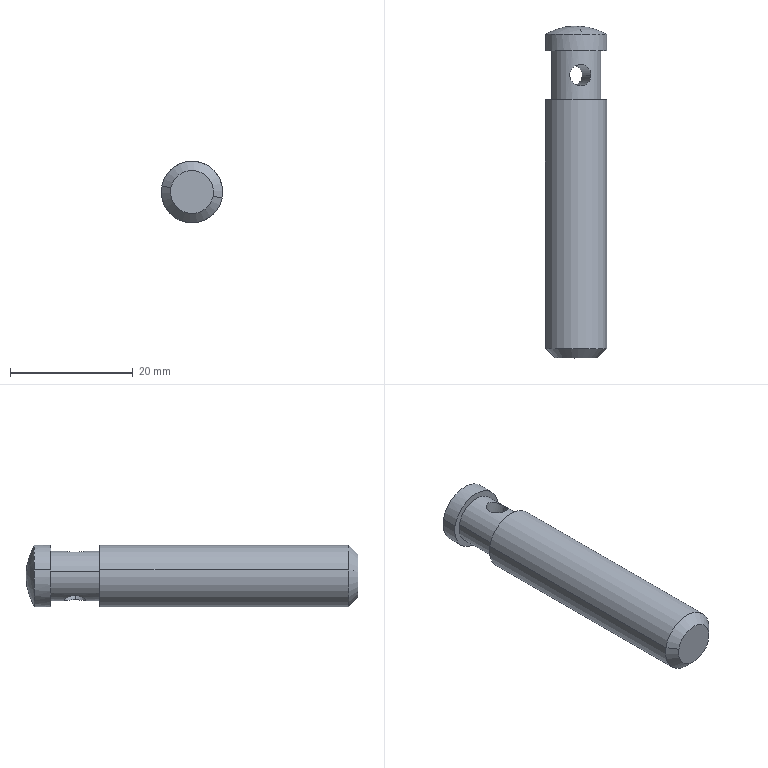Component | SolidWorks | JB_T8026.4-1999AdjustingSupportM10_40-3 | 1 solid | 15 faces | box 10 x 54 x 10 mm | volume 3857 mm3 | cylinder 8 | plane 3 | cone 2 | sphere 2 | commonest cylinder face diameters 10 x4 3.5 x2 8 x2
STEP:
#1=CARTESIAN_POINT('',(-4.944,8.292,0.1254));
#2=VERTEX_POINT('',#1);
#3=CARTESIAN_POINT('',(-5.079,8.292,0.1523));
#4=VERTEX_POINT('',#3);
#5=CARTESIAN_POINT('',(-4.944,8.292,0.1254));
#6=CARTESIAN_POINT('',(-4.944,8.296,0.1254));
#7=CARTESIAN_POINT('',(-4.945,8.301,0.1257));
#8=CARTESIAN_POINT('',(-4.946,8.31,0.1269));
#9=CARTESIAN_POINT('',(-4.947,8.314,0.1278));
#10=CARTESIAN_POINT('',(-4.952,8.326,0.1311));
#11=CARTESIAN_POINT('',(-4.957,8.334,0.1341));
#12=CARTESIAN_POINT('',(-4.968,8.347,0.1406));
#13=CARTESIAN_POINT('',(-4.975,8.352,0.144));
#14=CARTESIAN_POINT('',(-4.987,8.357,0.1485));
#15=CARTESIAN_POINT('',(-4.991,8.358,0.15));
#16=CARTESIAN_POINT('',(-5.,8.36,0.1525));
#17=CARTESIAN_POINT('',(-5.004,8.36,0.1535));
#18=CARTESIAN_POINT('',(-5.013,8.36,0.1553));
#19=CARTESIAN_POINT('',(-5.018,8.36,0.156));
#20=CARTESIAN_POINT('',(-5.026,8.358,0.157));
#21=CARTESIAN_POINT('',(-5.031,8.357,0.1573));
#22=CARTESIAN_POINT('',(-5.039,8.353,0.1575));
#23=CARTESIAN_POINT('',(-5.043,8.351,0.1575));
#24=CARTESIAN_POINT('',(-5.051,8.346,0.1571));
#25=CARTESIAN_POINT('',(-5.055,8.343,0.1568));
#26=CARTESIAN_POINT('',(-5.061,8.337,0.156));
#27=CARTESIAN_POINT('',(-5.064,8.334,0.1555));
#28=CARTESIAN_POINT('',(-5.069,8.326,0.1546));
#29=CARTESIAN_POINT('',(-5.072,8.322,0.1541));
#30=CARTESIAN_POINT('',(-5.077,8.31,0.1529));
#31=CARTESIAN_POINT('',(-5.079,8.301,0.1523));
#32=CARTESIAN_POINT('',(-5.079,8.292,0.1523));
#33=B_SPLINE_CURVE_WITH_KNOTS('',3,(#5,#6,#7,#8,#9,#10,#11,#12,#13,#14,#15,#16,#17,#18,#19,#20,#21,#22,#23,#24,#25,#26,#27,#28,#29,#30,#31,#32),.UNSPECIFIED.,.F.,.F.,(4,2,2,2,2,2,2,2,2,2,2,2,2,4),(0.,0.0003464,0.0006927,0.001385,0.002078,0.002425,0.002771,0.003117,0.003464,0.00381,0.004156,0.004503,0.004849,0.005542),.UNSPECIFIED.);
#34=EDGE_CURVE('',#2,#4,#33,.T.);
#35=ORIENTED_EDGE('',*,*,#34,.T.);
#36=CARTESIAN_POINT('',(-5.135,8.292,-0.1254));
#37=VERTEX_POINT('',#36);
#38=CARTESIAN_POINT('',(-5.068,8.292,0.2065));
#39=DIRECTION('',(-0.1956,0.,-0.9807));
#40=VECTOR('',#39,39.37);
#41=LINE('',#38,#40);
#42=EDGE_CURVE('',#4,#37,#41,.T.);
#43=ORIENTED_EDGE('',*,*,#42,.T.);
#44=CARTESIAN_POINT('',(-4.999,8.292,-0.1523));
#45=VERTEX_POINT('',#44);
#46=CARTESIAN_POINT('',(-5.135,8.292,-0.1254));
#47=CARTESIAN_POINT('',(-5.135,8.296,-0.1254));
#48=CARTESIAN_POINT('',(-5.134,8.301,-0.1257));
#49=CARTESIAN_POINT('',(-5.133,8.31,-0.1269));
#50=CARTESIAN_POINT('',(-5.131,8.314,-0.1278));
#51=CARTESIAN_POINT('',(-5.127,8.326,-0.1311));
#52=CARTESIAN_POINT('',(-5.122,8.334,-0.1341));
#53=CARTESIAN_POINT('',(-5.114,8.343,-0.139));
#54=CARTESIAN_POINT('',(-5.11,8.346,-0.1406));
#55=CARTESIAN_POINT('',(-5.103,8.351,-0.1439));
#56=CARTESIAN_POINT('',(-5.1,8.353,-0.1455));
#57=CARTESIAN_POINT('',(-5.092,8.357,-0.1485));
#58=CARTESIAN_POINT('',(-5.088,8.358,-0.1499));
#59=CARTESIAN_POINT('',(-5.079,8.36,-0.1524));
#60=CARTESIAN_POINT('',(-5.075,8.36,-0.1535));
#61=CARTESIAN_POINT('',(-5.061,8.36,-0.1562));
#62=CARTESIAN_POINT('',(-5.052,8.359,-0.1572));
#63=CARTESIAN_POINT('',(-5.039,8.353,-0.1575));
#64=CARTESIAN_POINT('',(-5.035,8.351,-0.1575));
#65=CARTESIAN_POINT('',(-5.028,8.346,-0.1571));
#66=CARTESIAN_POINT('',(-5.024,8.343,-0.1568));
#67=CARTESIAN_POINT('',(-5.014,8.334,-0.1556));
#68=CARTESIAN_POINT('',(-5.009,8.326,-0.1546));
#69=CARTESIAN_POINT('',(-5.003,8.314,-0.1533));
#70=CARTESIAN_POINT('',(-5.002,8.31,-0.153));
#71=CARTESIAN_POINT('',(-5.,8.301,-0.1525));
#72=CARTESIAN_POINT('',(-4.999,8.296,-0.1523));
#73=CARTESIAN_POINT('',(-4.999,8.292,-0.1523));
#74=B_SPLINE_CURVE_WITH_KNOTS('',3,(#46,#47,#48,#49,#50,#51,#52,#53,#54,#55,#56,#57,#58,#59,#60,#61,#62,#63,#64,#65,#66,#67,#68,#69,#70,#71,#72,#73),.UNSPECIFIED.,.F.,.F.,(4,2,2,2,2,2,2,2,2,2,2,2,2,4),(0.005542,0.005888,0.006234,0.006926,0.007272,0.007618,0.007964,0.00831,0.009002,0.009348,0.009694,0.01039,0.01073,0.01108),.UNSPECIFIED.);
#75=EDGE_CURVE('',#37,#45,#74,.T.);
#76=ORIENTED_EDGE('',*,*,#75,.T.);
#77=CARTESIAN_POINT('',(-4.933,8.292,0.1796));
#78=DIRECTION('',(-0.1956,0.,-0.9807));
#79=VECTOR('',#78,39.37);
#80=LINE('',#77,#79);
#81=EDGE_CURVE('',#2,#45,#80,.T.);
#82=ORIENTED_EDGE('',*,*,#81,.F.);
#83=EDGE_LOOP('',(#35,#43,#76,#82));
#84=FACE_OUTER_BOUND('',#83,.T.);
#85=CARTESIAN_POINT('',(-5.001,8.292,0.193));
#86=DIRECTION('',(-0.1956,0.,-0.9807));
#87=DIRECTION('',(0.9807,0.,-0.1956));
#88=AXIS2_PLACEMENT_3D('',#85,#86,#87);
#89=CYLINDRICAL_SURFACE('',#88,0.0689);
#90=ADVANCED_FACE('',(#84),#89,.F.);
#91=CARTESIAN_POINT('',(-5.175,6.481,0.02695));
#92=VERTEX_POINT('',#91);
#93=CARTESIAN_POINT('',(-4.904,6.481,-0.02695));
#94=VERTEX_POINT('',#93);
#95=CARTESIAN_POINT('',(-5.039,6.481,0.));
#96=DIRECTION('',(0.,-1.,0.));
#97=DIRECTION('',(-0.9807,0.,0.1956));
#98=AXIS2_PLACEMENT_3D('',#95,#96,#97);
#99=CIRCLE('',#98,0.1378);
#100=EDGE_CURVE('',#92,#94,#99,.T.);
#101=ORIENTED_EDGE('',*,*,#100,.F.);
#102=CARTESIAN_POINT('',(-5.232,6.54,0.0385));
#103=VERTEX_POINT('',#102);
#104=CARTESIAN_POINT('',(-5.232,6.54,0.0385));
#105=DIRECTION('',(-0.6935,0.7071,0.1383));
#106=VECTOR('',#105,39.37);
#107=LINE('',#104,#106);
#108=EDGE_CURVE('',#92,#103,#107,.T.);
#109=ORIENTED_EDGE('',*,*,#108,.T.);
#110=CARTESIAN_POINT('',(-4.846,6.54,-0.0385));
#111=VERTEX_POINT('',#110);
#112=CARTESIAN_POINT('',(-5.039,6.54,0.));
#113=DIRECTION('',(0.,1.,0.));
#114=DIRECTION('',(-0.9807,0.,0.1956));
#115=AXIS2_PLACEMENT_3D('',#112,#113,#114);
#116=CIRCLE('',#115,0.1969);
#117=EDGE_CURVE('',#111,#103,#116,.T.);
#118=ORIENTED_EDGE('',*,*,#117,.F.);
#119=CARTESIAN_POINT('',(-4.846,6.54,-0.0385));
#120=DIRECTION('',(0.6935,0.7071,-0.1383));
#121=VECTOR('',#120,39.37);
#122=LINE('',#119,#121);
#123=EDGE_CURVE('',#94,#111,#122,.T.);
#124=ORIENTED_EDGE('',*,*,#123,.F.);
#125=EDGE_LOOP('',(#101,#109,#118,#124));
#126=FACE_OUTER_BOUND('',#125,.T.);
#127=CARTESIAN_POINT('',(-5.039,6.54,0.));
#128=DIRECTION('',(0.,1.,0.));
#129=DIRECTION('',(0.9807,0.,-0.1956));
#130=AXIS2_PLACEMENT_3D('',#127,#128,#129);
#131=CONICAL_SURFACE('',#130,0.1969,0.7854);
#132=ADVANCED_FACE('',(#126),#131,.T.);
#133=ORIENTED_EDGE('',*,*,#117,.T.);
#134=CARTESIAN_POINT('',(-5.232,8.134,0.0385));
#135=VERTEX_POINT('',#134);
#136=CARTESIAN_POINT('',(-5.232,10.321,0.0385));
#137=DIRECTION('',(0.,1.,0.));
#138=VECTOR('',#137,39.37);
#139=LINE('',#136,#138);
#140=EDGE_CURVE('',#103,#135,#139,.T.);
#141=ORIENTED_EDGE('',*,*,#140,.T.);
#142=CARTESIAN_POINT('',(-4.846,8.134,-0.0385));
#143=VERTEX_POINT('',#142);
#144=CARTESIAN_POINT('',(-5.039,8.134,0.));
#145=DIRECTION('',(0.,1.,0.));
#146=DIRECTION('',(0.9807,0.,-0.1956));
#147=AXIS2_PLACEMENT_3D('',#144,#145,#146);
#148=CIRCLE('',#147,0.1969);
#149=EDGE_CURVE('',#143,#135,#148,.T.);
#150=ORIENTED_EDGE('',*,*,#149,.F.);
#151=CARTESIAN_POINT('',(-4.846,10.321,-0.0385));
#152=DIRECTION('',(0.,1.,0.));
#153=VECTOR('',#152,39.37);
#154=LINE('',#151,#153);
#155=EDGE_CURVE('',#111,#143,#154,.T.);
#156=ORIENTED_EDGE('',*,*,#155,.F.);
#157=EDGE_LOOP('',(#133,#141,#150,#156));
#158=FACE_OUTER_BOUND('',#157,.T.);
#159=CARTESIAN_POINT('',(-5.039,10.321,0.));
#160=DIRECTION('',(0.,1.,0.));
#161=DIRECTION('',(0.9807,0.,-0.1956));
#162=AXIS2_PLACEMENT_3D('',#159,#160,#161);
#163=CYLINDRICAL_SURFACE('',#162,0.1969);
#164=ADVANCED_FACE('',(#158),#163,.T.);
#165=CARTESIAN_POINT('',(-4.999,8.292,-0.1523));
#166=CARTESIAN_POINT('',(-4.999,8.287,-0.1523));
#167=CARTESIAN_POINT('',(-5.,8.282,-0.1525));
#168=CARTESIAN_POINT('',(-5.002,8.274,-0.153));
#169=CARTESIAN_POINT('',(-5.003,8.269,-0.1533));
#170=CARTESIAN_POINT('',(-5.009,8.257,-0.1546));
#171=CARTESIAN_POINT('',(-5.014,8.249,-0.1556));
#172=CARTESIAN_POINT('',(-5.027,8.237,-0.1572));
#173=CARTESIAN_POINT('',(-5.035,8.231,-0.1577));
#174=CARTESIAN_POINT('',(-5.048,8.226,-0.1573));
#175=CARTESIAN_POINT('',(-5.052,8.225,-0.157));
#176=CARTESIAN_POINT('',(-5.061,8.223,-0.156));
#177=CARTESIAN_POINT('',(-5.066,8.223,-0.1553));
#178=CARTESIAN_POINT('',(-5.075,8.223,-0.1536));
#179=CARTESIAN_POINT('',(-5.079,8.223,-0.1525));
#180=CARTESIAN_POINT('',(-5.088,8.225,-0.15));
#181=CARTESIAN_POINT('',(-5.092,8.226,-0.1485));
#182=CARTESIAN_POINT('',(-5.1,8.23,-0.1455));
#183=CARTESIAN_POINT('',(-5.103,8.232,-0.1439));
#184=CARTESIAN_POINT('',(-5.11,8.237,-0.1406));
#185=CARTESIAN_POINT('',(-5.114,8.24,-0.1389));
#186=CARTESIAN_POINT('',(-5.119,8.246,-0.1357));
#187=CARTESIAN_POINT('',(-5.122,8.249,-0.1341));
#188=CARTESIAN_POINT('',(-5.126,8.257,-0.1312));
#189=CARTESIAN_POINT('',(-5.128,8.261,-0.1299));
#190=CARTESIAN_POINT('',(-5.133,8.273,-0.1267));
#191=CARTESIAN_POINT('',(-5.135,8.282,-0.1254));
#192=CARTESIAN_POINT('',(-5.135,8.292,-0.1254));
#193=B_SPLINE_CURVE_WITH_KNOTS('',3,(#165,#166,#167,#168,#169,#170,#171,#172,#173,#174,#175,#176,#177,#178,#179,#180,#181,#182,#183,#184,#185,#186,#187,#188,#189,#190,#191,#192),.UNSPECIFIED.,.F.,.F.,(4,2,2,2,2,2,2,2,2,2,2,2,2,4),(0.,0.0003464,0.0006927,0.001385,0.002078,0.002425,0.002771,0.003117,0.003464,0.00381,0.004156,0.004503,0.004849,0.005542),.UNSPECIFIED.);
#194=EDGE_CURVE('',#45,#37,#193,.T.);
#195=ORIENTED_EDGE('',*,*,#194,.F.);
#196=ORIENTED_EDGE('',*,*,#75,.F.);
#197=EDGE_LOOP('',(#195,#196));
#198=FACE_BOUND('',#197,.T.);
#199=CARTESIAN_POINT('',(-4.885,8.134,-0.0308));
#200=VERTEX_POINT('',#199);
#201=CARTESIAN_POINT('',(-5.194,8.134,0.0308));
#202=VERTEX_POINT('',#201);
#203=CARTESIAN_POINT('',(-5.039,8.134,0.));
#204=DIRECTION('',(0.,1.,0.));
#205=DIRECTION('',(0.9807,0.,-0.1956));
#206=AXIS2_PLACEMENT_3D('',#203,#204,#205);
#207=CIRCLE('',#206,0.1575);
#208=EDGE_CURVE('',#200,#202,#207,.T.);
#209=ORIENTED_EDGE('',*,*,#208,.T.);
#210=CARTESIAN_POINT('',(-5.194,8.449,0.0308));
#211=VERTEX_POINT('',#210);
#212=CARTESIAN_POINT('',(-5.194,10.321,0.0308));
#213=DIRECTION('',(0.,1.,0.));
#214=VECTOR('',#213,39.37);
#215=LINE('',#212,#214);
#216=EDGE_CURVE('',#202,#211,#215,.T.);
#217=ORIENTED_EDGE('',*,*,#216,.T.);
#218=CARTESIAN_POINT('',(-4.885,8.449,-0.0308));
#219=VERTEX_POINT('',#218);
#220=CARTESIAN_POINT('',(-5.039,8.449,0.));
#221=DIRECTION('',(0.,1.,0.));
#222=DIRECTION('',(0.9807,0.,-0.1956));
#223=AXIS2_PLACEMENT_3D('',#220,#221,#222);
#224=CIRCLE('',#223,0.1575);
#225=EDGE_CURVE('',#219,#211,#224,.T.);
#226=ORIENTED_EDGE('',*,*,#225,.F.);
#227=CARTESIAN_POINT('',(-4.885,10.321,-0.0308));
#228=DIRECTION('',(0.,1.,0.));
#229=VECTOR('',#228,39.37);
#230=LINE('',#227,#229);
#231=EDGE_CURVE('',#200,#219,#230,.T.);
#232=ORIENTED_EDGE('',*,*,#231,.F.);
#233=EDGE_LOOP('',(#209,#217,#226,#232));
#234=FACE_OUTER_BOUND('',#233,.T.);
#235=CARTESIAN_POINT('',(-5.039,10.321,0.));
#236=DIRECTION('',(0.,1.,0.));
#237=DIRECTION('',(0.9807,0.,-0.1956));
#238=AXIS2_PLACEMENT_3D('',#235,#236,#237);
#239=CYLINDRICAL_SURFACE('',#238,0.1575);
#240=ADVANCED_FACE('',(#198,#234),#239,.T.);
#241=CARTESIAN_POINT('',(-4.846,8.449,-0.0385));
#242=VERTEX_POINT('',#241);
#243=CARTESIAN_POINT('',(-5.232,8.449,0.0385));
#244=VERTEX_POINT('',#243);
#245=CARTESIAN_POINT('',(-5.039,8.449,0.));
#246=DIRECTION('',(0.,1.,0.));
#247=DIRECTION('',(0.9807,0.,-0.1956));
#248=AXIS2_PLACEMENT_3D('',#245,#246,#247);
#249=CIRCLE('',#248,0.1969);
#250=EDGE_CURVE('',#242,#244,#249,.T.);
#251=ORIENTED_EDGE('',*,*,#250,.T.);
#252=CARTESIAN_POINT('',(-5.232,8.554,0.0385));
#253=VERTEX_POINT('',#252);
#254=CARTESIAN_POINT('',(-5.232,10.321,0.0385));
#255=DIRECTION('',(0.,1.,0.));
#256=VECTOR('',#255,39.37);
#257=LINE('',#254,#256);
#258=EDGE_CURVE('',#244,#253,#257,.T.);
#259=ORIENTED_EDGE('',*,*,#258,.T.);
#260=CARTESIAN_POINT('',(-5.078,8.554,-0.193));
#261=VERTEX_POINT('',#260);
#262=CARTESIAN_POINT('',(-5.039,8.554,0.));
#263=DIRECTION('',(0.,1.,0.));
#264=DIRECTION('',(0.9807,0.,-0.1956));
#265=AXIS2_PLACEMENT_3D('',#262,#263,#264);
#266=CIRCLE('',#265,0.1969);
#267=EDGE_CURVE('',#261,#253,#266,.T.);
#268=ORIENTED_EDGE('',*,*,#267,.F.);
#269=CARTESIAN_POINT('',(-4.846,8.554,-0.0385));
#270=VERTEX_POINT('',#269);
#271=CARTESIAN_POINT('',(-5.039,8.554,0.));
#272=DIRECTION('',(0.,1.,0.));
#273=DIRECTION('',(0.9807,0.,-0.1956));
#274=AXIS2_PLACEMENT_3D('',#271,#272,#273);
#275=CIRCLE('',#274,0.1969);
#276=EDGE_CURVE('',#270,#261,#275,.T.);
#277=ORIENTED_EDGE('',*,*,#276,.F.);
#278=CARTESIAN_POINT('',(-4.846,10.321,-0.0385));
#279=DIRECTION('',(0.,1.,0.));
#280=VECTOR('',#279,39.37);
#281=LINE('',#278,#280);
#282=EDGE_CURVE('',#242,#270,#281,.T.);
#283=ORIENTED_EDGE('',*,*,#282,.F.);
#284=EDGE_LOOP('',(#251,#259,#268,#277,#283));
#285=FACE_OUTER_BOUND('',#284,.T.);
#286=CARTESIAN_POINT('',(-5.039,10.321,0.));
#287=DIRECTION('',(0.,1.,0.));
#288=DIRECTION('',(0.9807,0.,-0.1956));
#289=AXIS2_PLACEMENT_3D('',#286,#287,#288);
#290=CYLINDRICAL_SURFACE('',#289,0.1969);
#291=ADVANCED_FACE('',(#285),#290,.T.);
#292=ORIENTED_EDGE('',*,*,#267,.T.);
#293=CARTESIAN_POINT('',(-5.001,8.554,0.193));
#294=VERTEX_POINT('',#293);
#295=CARTESIAN_POINT('',(-5.039,8.554,0.));
#296=DIRECTION('',(0.,1.,0.));
#297=DIRECTION('',(0.9807,0.,-0.1956));
#298=AXIS2_PLACEMENT_3D('',#295,#296,#297);
#299=CIRCLE('',#298,0.1969);
#300=EDGE_CURVE('',#253,#294,#299,.T.);
#301=ORIENTED_EDGE('',*,*,#300,.T.);
#302=CARTESIAN_POINT('',(-5.039,8.607,-0.));
#303=VERTEX_POINT('',#302);
#304=CARTESIAN_POINT('',(-5.039,8.213,0.));
#305=DIRECTION('',(-0.9807,0.,0.1956));
#306=DIRECTION('',(0.1956,0.,0.9807));
#307=AXIS2_PLACEMENT_3D('',#304,#305,#306);
#308=CIRCLE('',#307,0.3937);
#309=EDGE_CURVE('',#294,#303,#308,.T.);
#310=ORIENTED_EDGE('',*,*,#309,.T.);
#311=CARTESIAN_POINT('',(-5.039,8.213,0.));
#312=DIRECTION('',(0.9807,0.,-0.1956));
#313=DIRECTION('',(-0.1956,0.,-0.9807));
#314=AXIS2_PLACEMENT_3D('',#311,#312,#313);
#315=CIRCLE('',#314,0.3937);
#316=EDGE_CURVE('',#261,#303,#315,.T.);
#317=ORIENTED_EDGE('',*,*,#316,.F.);
#318=EDGE_LOOP('',(#292,#301,#310,#317));
#319=FACE_OUTER_BOUND('',#318,.T.);
#320=CARTESIAN_POINT('',(-5.039,8.213,0.));
#321=DIRECTION('',(-0.9807,0.,0.1956));
#322=DIRECTION('',(-0.1956,0.,-0.9807));
#323=AXIS2_PLACEMENT_3D('',#320,#321,#322);
#324=SPHERICAL_SURFACE('',#323,0.3937);
#325=ADVANCED_FACE('',(#319),#324,.T.);
#326=CARTESIAN_POINT('',(-5.039,6.481,0.));
#327=DIRECTION('',(0.,-1.,0.));
#328=DIRECTION('',(-0.9807,0.,0.1956));
#329=AXIS2_PLACEMENT_3D('',#326,#327,#328);
#330=CIRCLE('',#329,0.1378);
#331=EDGE_CURVE('',#94,#92,#330,.T.);
#332=ORIENTED_EDGE('',*,*,#331,.T.);
#333=ORIENTED_EDGE('',*,*,#100,.T.);
#334=EDGE_LOOP('',(#332,#333));
#335=FACE_OUTER_BOUND('',#334,.T.);
#336=CARTESIAN_POINT('',(-5.012,6.481,0.1351));
#337=DIRECTION('',(0.,-1.,0.));
#338=DIRECTION('',(-0.9807,0.,0.1956));
#339=AXIS2_PLACEMENT_3D('',#336,#337,#338);
#340=PLANE('',#339);
#341=ADVANCED_FACE('',(#335),#340,.T.);
#342=ORIENTED_EDGE('',*,*,#309,.F.);
#343=CARTESIAN_POINT('',(-5.039,8.554,0.));
#344=DIRECTION('',(0.,1.,0.));
#345=DIRECTION('',(0.9807,0.,-0.1956));
#346=AXIS2_PLACEMENT_3D('',#343,#344,#345);
#347=CIRCLE('',#346,0.1969);
#348=EDGE_CURVE('',#294,#270,#347,.T.);
#349=ORIENTED_EDGE('',*,*,#348,.T.);
#350=ORIENTED_EDGE('',*,*,#276,.T.);
#351=ORIENTED_EDGE('',*,*,#316,.T.);
#352=EDGE_LOOP('',(#342,#349,#350,#351));
#353=FACE_OUTER_BOUND('',#352,.T.);
#354=CARTESIAN_POINT('',(-5.039,8.213,0.));
#355=DIRECTION('',(-0.9807,0.,0.1956));
#356=DIRECTION('',(-0.1956,0.,-0.9807));
#357=AXIS2_PLACEMENT_3D('',#354,#355,#356);
#358=SPHERICAL_SURFACE('',#357,0.3937);
#359=ADVANCED_FACE('',(#353),#358,.T.);
#360=ORIENTED_EDGE('',*,*,#258,.F.);
#361=CARTESIAN_POINT('',(-5.039,8.449,0.));
#362=DIRECTION('',(0.,1.,0.));
#363=DIRECTION('',(0.9807,0.,-0.1956));
#364=AXIS2_PLACEMENT_3D('',#361,#362,#363);
#365=CIRCLE('',#364,0.1969);
#366=EDGE_CURVE('',#244,#242,#365,.T.);
#367=ORIENTED_EDGE('',*,*,#366,.T.);
#368=ORIENTED_EDGE('',*,*,#282,.T.);
#369=ORIENTED_EDGE('',*,*,#348,.F.);
#370=ORIENTED_EDGE('',*,*,#300,.F.);
#371=EDGE_LOOP('',(#360,#367,#368,#369,#370));
#372=FACE_OUTER_BOUND('',#371,.T.);
#373=CARTESIAN_POINT('',(-5.039,10.321,0.));
#374=DIRECTION('',(0.,1.,0.));
#375=DIRECTION('',(0.9807,0.,-0.1956));
#376=AXIS2_PLACEMENT_3D('',#373,#374,#375);
#377=CYLINDRICAL_SURFACE('',#376,0.1969);
#378=ADVANCED_FACE('',(#372),#377,.T.);
#379=ORIENTED_EDGE('',*,*,#225,.T.);
#380=CARTESIAN_POINT('',(-5.039,8.449,0.));
#381=DIRECTION('',(0.,1.,0.));
#382=DIRECTION('',(0.9807,0.,-0.1956));
#383=AXIS2_PLACEMENT_3D('',#380,#381,#382);
#384=CIRCLE('',#383,0.1575);
#385=EDGE_CURVE('',#211,#219,#384,.T.);
#386=ORIENTED_EDGE('',*,*,#385,.T.);
#387=EDGE_LOOP('',(#379,#386));
#388=FACE_BOUND('',#387,.T.);
#389=ORIENTED_EDGE('',*,*,#250,.F.);
#390=ORIENTED_EDGE('',*,*,#366,.F.);
#391=EDGE_LOOP('',(#389,#390));
#392=FACE_OUTER_BOUND('',#391,.T.);
#393=CARTESIAN_POINT('',(-5.001,8.449,0.193));
#394=DIRECTION('',(0.,-1.,0.));
#395=DIRECTION('',(-0.9807,0.,0.1956));
#396=AXIS2_PLACEMENT_3D('',#393,#394,#395);
#397=PLANE('',#396);
#398=ADVANCED_FACE('',(#388,#392),#397,.T.);
#399=ORIENTED_EDGE('',*,*,#216,.F.);
#400=CARTESIAN_POINT('',(-5.039,8.134,0.));
#401=DIRECTION('',(0.,1.,0.));
#402=DIRECTION('',(0.9807,0.,-0.1956));
#403=AXIS2_PLACEMENT_3D('',#400,#401,#402);
#404=CIRCLE('',#403,0.1575);
#405=EDGE_CURVE('',#202,#200,#404,.T.);
#406=ORIENTED_EDGE('',*,*,#405,.T.);
#407=ORIENTED_EDGE('',*,*,#231,.T.);
#408=ORIENTED_EDGE('',*,*,#385,.F.);
#409=EDGE_LOOP('',(#399,#406,#407,#408));
#410=FACE_OUTER_BOUND('',#409,.T.);
#411=ORIENTED_EDGE('',*,*,#34,.F.);
#412=CARTESIAN_POINT('',(-5.079,8.292,0.1523));
#413=CARTESIAN_POINT('',(-5.079,8.287,0.1523));
#414=CARTESIAN_POINT('',(-5.079,8.282,0.1525));
#415=CARTESIAN_POINT('',(-5.077,8.273,0.153));
#416=CARTESIAN_POINT('',(-5.075,8.269,0.1533));
#417=CARTESIAN_POINT('',(-5.07,8.257,0.1546));
#418=CARTESIAN_POINT('',(-5.064,8.249,0.1556));
#419=CARTESIAN_POINT('',(-5.055,8.24,0.1568));
#420=CARTESIAN_POINT('',(-5.051,8.237,0.1571));
#421=CARTESIAN_POINT('',(-5.043,8.232,0.1575));
#422=CARTESIAN_POINT('',(-5.039,8.23,0.1575));
#423=CARTESIAN_POINT('',(-5.031,8.226,0.1573));
#424=CARTESIAN_POINT('',(-5.027,8.225,0.157));
#425=CARTESIAN_POINT('',(-5.018,8.223,0.156));
#426=CARTESIAN_POINT('',(-5.013,8.223,0.1553));
#427=CARTESIAN_POINT('',(-5.,8.223,0.1527));
#428=CARTESIAN_POINT('',(-4.991,8.225,0.1501));
#429=CARTESIAN_POINT('',(-4.979,8.23,0.1455));
#430=CARTESIAN_POINT('',(-4.975,8.232,0.1439));
#431=CARTESIAN_POINT('',(-4.968,8.237,0.1406));
#432=CARTESIAN_POINT('',(-4.965,8.24,0.139));
#433=CARTESIAN_POINT('',(-4.956,8.249,0.1341));
#434=CARTESIAN_POINT('',(-4.952,8.257,0.1311));
#435=CARTESIAN_POINT('',(-4.947,8.269,0.1278));
#436=CARTESIAN_POINT('',(-4.946,8.273,0.1269));
#437=CARTESIAN_POINT('',(-4.945,8.282,0.1257));
#438=CARTESIAN_POINT('',(-4.944,8.287,0.1254));
#439=CARTESIAN_POINT('',(-4.944,8.292,0.1254));
#440=B_SPLINE_CURVE_WITH_KNOTS('',3,(#412,#413,#414,#415,#416,#417,#418,#419,#420,#421,#422,#423,#424,#425,#426,#427,#428,#429,#430,#431,#432,#433,#434,#435,#436,#437,#438,#439),.UNSPECIFIED.,.F.,.F.,(4,2,2,2,2,2,2,2,2,2,2,2,2,4),(0.005542,0.005888,0.006234,0.006926,0.007272,0.007618,0.007964,0.00831,0.009002,0.009348,0.009694,0.01039,0.01073,0.01108),.UNSPECIFIED.);
#441=EDGE_CURVE('',#4,#2,#440,.T.);
#442=ORIENTED_EDGE('',*,*,#441,.F.);
#443=EDGE_LOOP('',(#411,#442));
#444=FACE_BOUND('',#443,.T.);
#445=CARTESIAN_POINT('',(-5.039,10.321,0.));
#446=DIRECTION('',(0.,1.,0.));
#447=DIRECTION('',(0.9807,0.,-0.1956));
#448=AXIS2_PLACEMENT_3D('',#445,#446,#447);
#449=CYLINDRICAL_SURFACE('',#448,0.1575);
#450=ADVANCED_FACE('',(#410,#444),#449,.T.);
#451=ORIENTED_EDGE('',*,*,#149,.T.);
#452=CARTESIAN_POINT('',(-5.039,8.134,0.));
#453=DIRECTION('',(0.,1.,0.));
#454=DIRECTION('',(0.9807,0.,-0.1956));
#455=AXIS2_PLACEMENT_3D('',#452,#453,#454);
#456=CIRCLE('',#455,0.1969);
#457=EDGE_CURVE('',#135,#143,#456,.T.);
#458=ORIENTED_EDGE('',*,*,#457,.T.);
#459=EDGE_LOOP('',(#451,#458));
#460=FACE_OUTER_BOUND('',#459,.T.);
#461=ORIENTED_EDGE('',*,*,#208,.F.);
#462=ORIENTED_EDGE('',*,*,#405,.F.);
#463=EDGE_LOOP('',(#461,#462));
#464=FACE_BOUND('',#463,.T.);
#465=CARTESIAN_POINT('',(-5.009,8.134,0.1544));
#466=DIRECTION('',(0.,1.,0.));
#467=DIRECTION('',(0.9807,0.,-0.1956));
#468=AXIS2_PLACEMENT_3D('',#465,#466,#467);
#469=PLANE('',#468);
#470=ADVANCED_FACE('',(#460,#464),#469,.T.);
#471=ORIENTED_EDGE('',*,*,#140,.F.);
#472=CARTESIAN_POINT('',(-5.039,6.54,0.));
#473=DIRECTION('',(0.,1.,0.));
#474=DIRECTION('',(-0.9807,0.,0.1956));
#475=AXIS2_PLACEMENT_3D('',#472,#473,#474);
#476=CIRCLE('',#475,0.1969);
#477=EDGE_CURVE('',#103,#111,#476,.T.);
#478=ORIENTED_EDGE('',*,*,#477,.T.);
#479=ORIENTED_EDGE('',*,*,#155,.T.);
#480=ORIENTED_EDGE('',*,*,#457,.F.);
#481=EDGE_LOOP('',(#471,#478,#479,#480));
#482=FACE_OUTER_BOUND('',#481,.T.);
#483=CARTESIAN_POINT('',(-5.039,10.321,0.));
#484=DIRECTION('',(0.,1.,0.));
#485=DIRECTION('',(0.9807,0.,-0.1956));
#486=AXIS2_PLACEMENT_3D('',#483,#484,#485);
#487=CYLINDRICAL_SURFACE('',#486,0.1969);
#488=ADVANCED_FACE('',(#482),#487,.T.);
#489=ORIENTED_EDGE('',*,*,#108,.F.);
#490=ORIENTED_EDGE('',*,*,#331,.F.);
#491=ORIENTED_EDGE('',*,*,#123,.T.);
#492=ORIENTED_EDGE('',*,*,#477,.F.);
#493=EDGE_LOOP('',(#489,#490,#491,#492));
#494=FACE_OUTER_BOUND('',#493,.T.);
#495=CARTESIAN_POINT('',(-5.039,6.54,0.));
#496=DIRECTION('',(0.,1.,0.));
#497=DIRECTION('',(0.9807,0.,-0.1956));
#498=AXIS2_PLACEMENT_3D('',#495,#496,#497);
#499=CONICAL_SURFACE('',#498,0.1969,0.7854);
#500=ADVANCED_FACE('',(#494),#499,.T.);
#501=ORIENTED_EDGE('',*,*,#42,.F.);
#502=ORIENTED_EDGE('',*,*,#441,.T.);
#503=ORIENTED_EDGE('',*,*,#81,.T.);
#504=ORIENTED_EDGE('',*,*,#194,.T.);
#505=EDGE_LOOP('',(#501,#502,#503,#504));
#506=FACE_OUTER_BOUND('',#505,.T.);
#507=CARTESIAN_POINT('',(-5.001,8.292,0.193));
#508=DIRECTION('',(-0.1956,0.,-0.9807));
#509=DIRECTION('',(0.9807,0.,-0.1956));
#510=AXIS2_PLACEMENT_3D('',#507,#508,#509);
#511=CYLINDRICAL_SURFACE('',#510,0.0689);
#512=ADVANCED_FACE('',(#506),#511,.F.);
#513=CLOSED_SHELL('',(#90,#132,#164,#240,#291,#325,#341,#359,#378,#398,#450,#470,#488,#500,#512));
#514=MANIFOLD_SOLID_BREP('',#513);
#515=CARTESIAN_POINT('',(0.,0.,0.));
#516=DIRECTION('',(0.,0.,1.));
#517=DIRECTION('',(1.,0.,0.));
#518=AXIS2_PLACEMENT_3D('',#515,#516,#517);
#519=(LENGTH_UNIT()NAMED_UNIT(*)SI_UNIT($,.METRE.));
#520=LENGTH_MEASURE_WITH_UNIT(LENGTH_MEASURE(0.0254),#519);
#521=DIMENSIONAL_EXPONENTS(1.,0.,0.,0.,0.,0.,0.);
#522=(CONVERSION_BASED_UNIT('',#520)LENGTH_UNIT()NAMED_UNIT(#521));
#523=UNCERTAINTY_MEASURE_WITH_UNIT(LENGTH_MEASURE(0.00001),#522,'','');
#524=(NAMED_UNIT(*)PLANE_ANGLE_UNIT()SI_UNIT($,.RADIAN.));
#525=(NAMED_UNIT(*)SI_UNIT($,.STERADIAN.)SOLID_ANGLE_UNIT());
#526=(GEOMETRIC_REPRESENTATION_CONTEXT(3)GLOBAL_UNCERTAINTY_ASSIGNED_CONTEXT((#523))GLOBAL_UNIT_ASSIGNED_CONTEXT((#522,#524,#525))REPRESENTATION_CONTEXT('',''));
#527=ADVANCED_BREP_SHAPE_REPRESENTATION('',(#514,#518),#526);
#528=COLOUR_RGB('',0.7922,0.8196,0.9333);
#529=FILL_AREA_STYLE_COLOUR('',#528);
#530=FILL_AREA_STYLE('',(#529));
#531=SURFACE_STYLE_FILL_AREA(#530);
#532=SURFACE_SIDE_STYLE('',(#531));
#533=SURFACE_STYLE_USAGE(.BOTH.,#532);
#534=PRESENTATION_STYLE_ASSIGNMENT((#533));
#535=STYLED_ITEM('',(#534),#514);
#536=(LENGTH_UNIT()NAMED_UNIT(*)SI_UNIT($,.METRE.));
#537=LENGTH_MEASURE_WITH_UNIT(LENGTH_MEASURE(0.0254),#536);
#538=DIMENSIONAL_EXPONENTS(1.,0.,0.,0.,0.,0.,0.);
#539=(CONVERSION_BASED_UNIT('',#537)LENGTH_UNIT()NAMED_UNIT(#538));
#540=UNCERTAINTY_MEASURE_WITH_UNIT(LENGTH_MEASURE(0.00001),#539,'','');
#541=(NAMED_UNIT(*)PLANE_ANGLE_UNIT()SI_UNIT($,.RADIAN.));
#542=(NAMED_UNIT(*)SI_UNIT($,.STERADIAN.)SOLID_ANGLE_UNIT());
#543=(GEOMETRIC_REPRESENTATION_CONTEXT(3)GLOBAL_UNCERTAINTY_ASSIGNED_CONTEXT((#540))GLOBAL_UNIT_ASSIGNED_CONTEXT((#539,#541,#542))REPRESENTATION_CONTEXT('',''));
#544=MECHANICAL_DESIGN_GEOMETRIC_PRESENTATION_REPRESENTATION('',(#535),#543);
#545=PRESENTATION_LAYER_ASSIGNMENT('','',(#535));